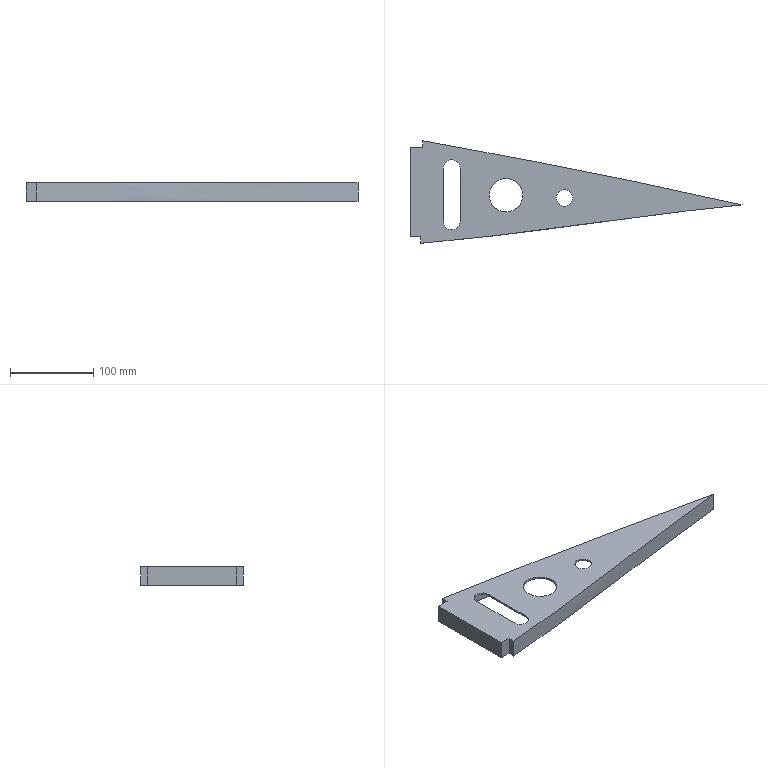Component | NX | REAR_RIB | 1 solid | 23 faces | volume 81872 mm3 | plane 15 | cylinder 4 | other 2 | spline 2 | commonest cylinder face diameters 20 x3 40 x1